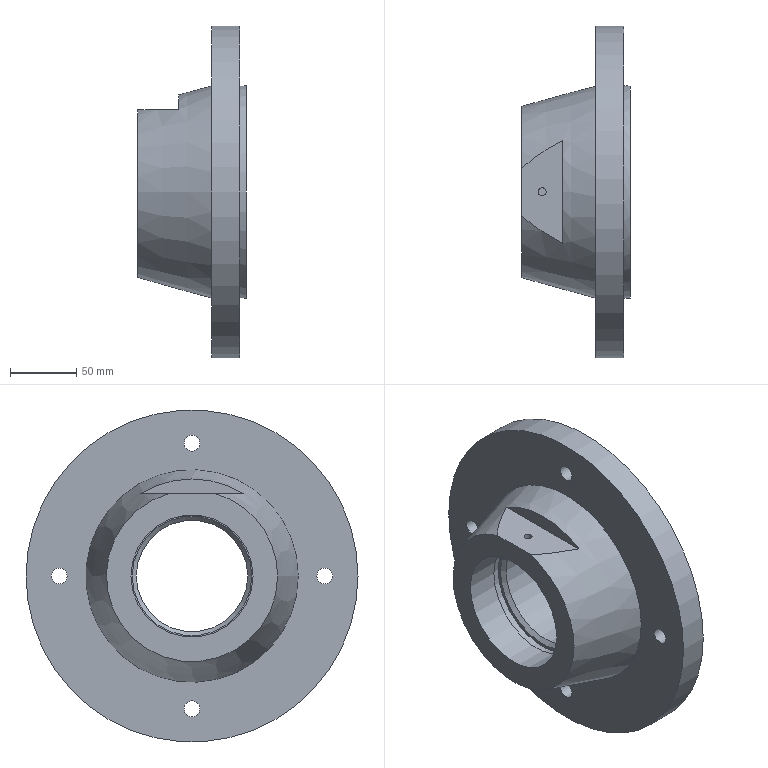Component | NX | ADAPTER_PLATE | 1 solid | 23 faces | volume 1519545 mm3 | cylinder 11 | plane 9 | cone 3 | commonest cylinder face diameters 12 x4 160 x1 250 x1 107 x1 84 x1 95 x1 92 x1 6 x1